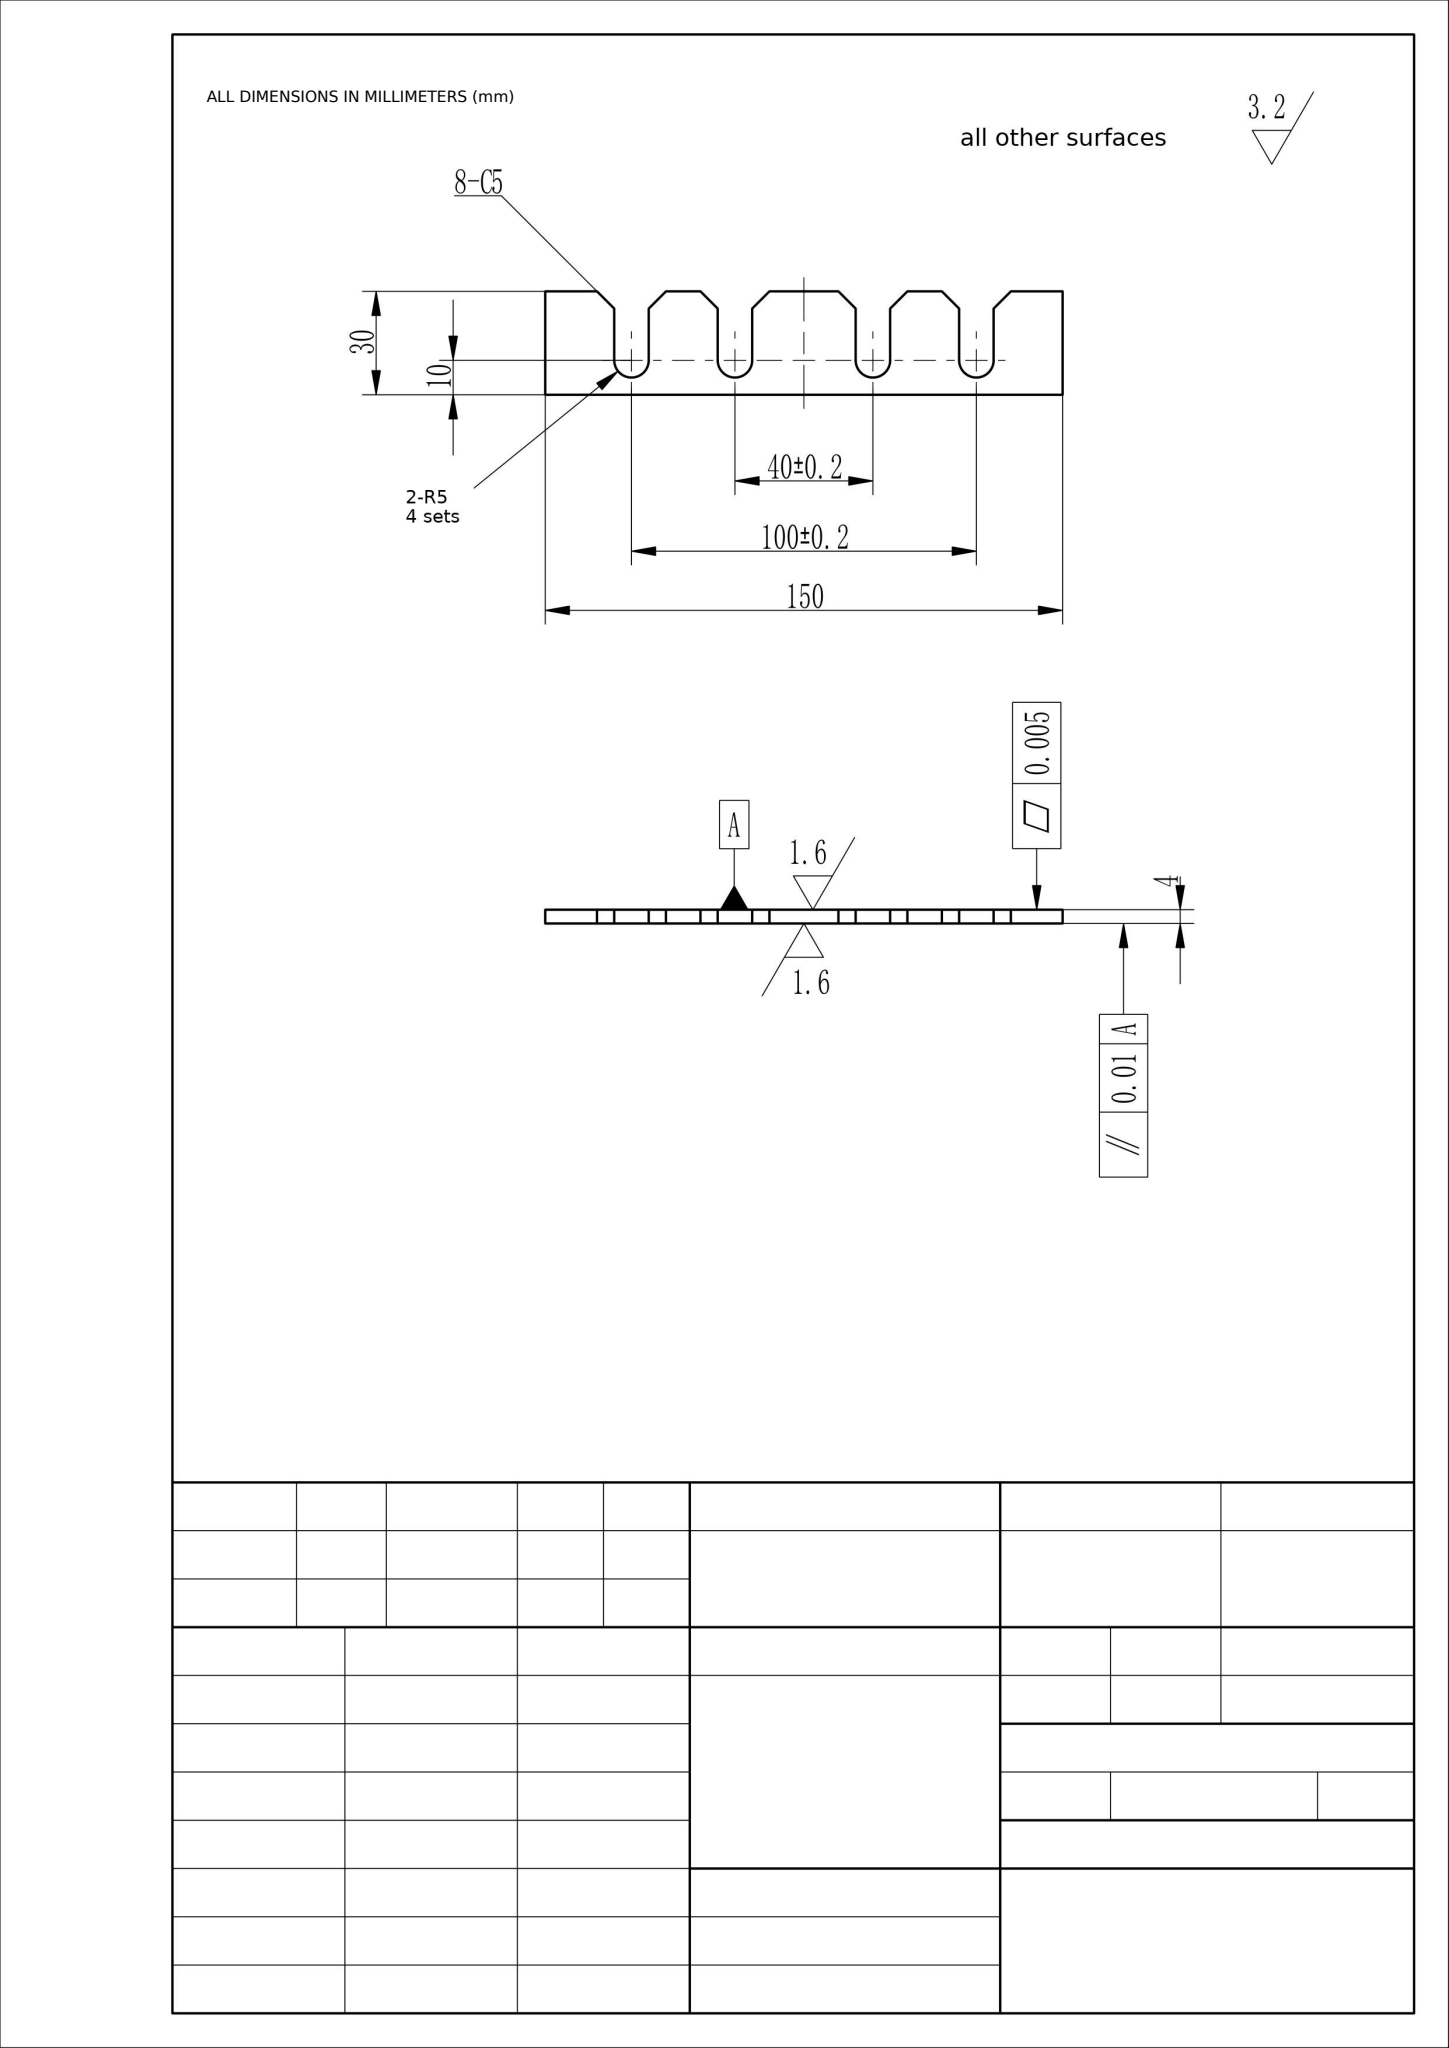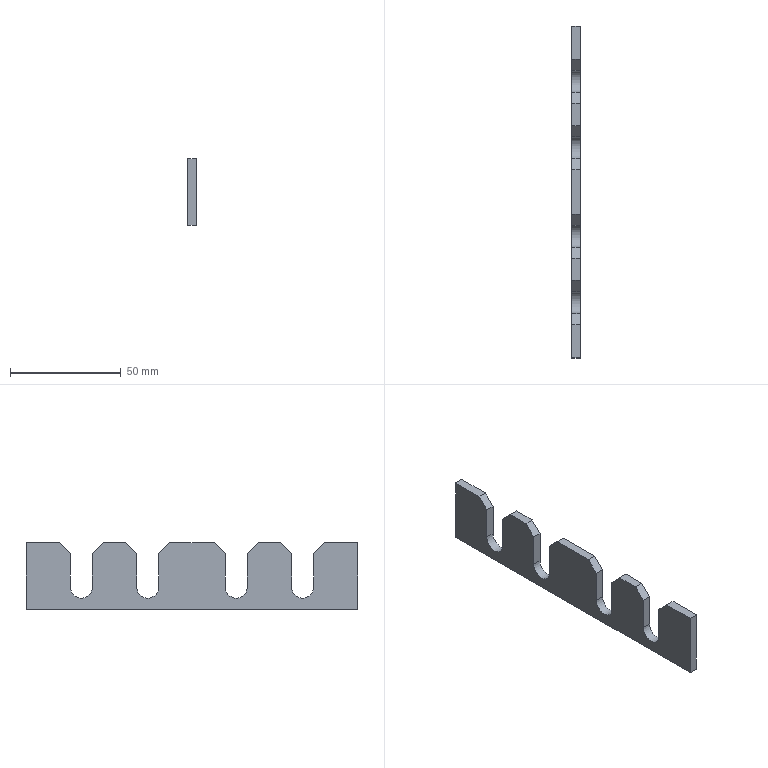Part | NX | mm | 1 solid | 30 faces | box 4 x 150 x 30 mm | volume 13772 mm3 | plane 26 | cylinder 4 | commonest cylinder face diameters 10 x4
STEP:
#1=CARTESIAN_POINT('',(0.,0.,0.));
#2=DIRECTION('',(0.,0.,1.));
#3=DIRECTION('',(1.,0.,0.));
#4=AXIS2_PLACEMENT_3D('',#1,#2,#3);
#5=(LENGTH_UNIT()NAMED_UNIT(*)SI_UNIT(.MILLI.,.METRE.));
#6=UNCERTAINTY_MEASURE_WITH_UNIT(LENGTH_MEASURE(0.00002),#5,'','');
#7=(NAMED_UNIT(*)PLANE_ANGLE_UNIT()SI_UNIT($,.RADIAN.));
#8=PLANE_ANGLE_MEASURE_WITH_UNIT(PLANE_ANGLE_MEASURE(0.01745),#7);
#9=DIMENSIONAL_EXPONENTS(0.,0.,0.,0.,0.,0.,0.);
#10=(CONVERSION_BASED_UNIT('',#8)NAMED_UNIT(#9)PLANE_ANGLE_UNIT());
#11=(NAMED_UNIT(*)SI_UNIT($,.STERADIAN.)SOLID_ANGLE_UNIT());
#12=(GEOMETRIC_REPRESENTATION_CONTEXT(3)GLOBAL_UNCERTAINTY_ASSIGNED_CONTEXT((#6))GLOBAL_UNIT_ASSIGNED_CONTEXT((#5,#10,#11))REPRESENTATION_CONTEXT('',''));
#13=SHAPE_REPRESENTATION('',(#4),#12);
#14=CARTESIAN_POINT('',(4.,-25.,-15.));
#15=VERTEX_POINT('',#14);
#16=CARTESIAN_POINT('',(4.,-25.,0.));
#17=VERTEX_POINT('',#16);
#18=CARTESIAN_POINT('',(4.,-25.,-15.));
#19=DIRECTION('',(0.,-0.,1.));
#20=VECTOR('',#19,1.);
#21=LINE('',#18,#20);
#22=EDGE_CURVE('',#15,#17,#21,.T.);
#23=ORIENTED_EDGE('',*,*,#22,.T.);
#24=CARTESIAN_POINT('',(4.,-30.,5.));
#25=VERTEX_POINT('',#24);
#26=CARTESIAN_POINT('',(4.,-12.5,-12.5));
#27=DIRECTION('',(0.,-0.7071,0.7071));
#28=VECTOR('',#27,1.);
#29=LINE('',#26,#28);
#30=EDGE_CURVE('',#17,#25,#29,.T.);
#31=ORIENTED_EDGE('',*,*,#30,.T.);
#32=CARTESIAN_POINT('',(4.,-40.,5.));
#33=VERTEX_POINT('',#32);
#34=CARTESIAN_POINT('',(4.,75.,5.));
#35=DIRECTION('',(0.,-1.,0.));
#36=VECTOR('',#35,1.);
#37=LINE('',#34,#36);
#38=EDGE_CURVE('',#25,#33,#37,.T.);
#39=ORIENTED_EDGE('',*,*,#38,.T.);
#40=CARTESIAN_POINT('',(4.,-45.,0.));
#41=VERTEX_POINT('',#40);
#42=CARTESIAN_POINT('',(4.,-22.5,22.5));
#43=DIRECTION('',(0.,-0.7071,-0.7071));
#44=VECTOR('',#43,1.);
#45=LINE('',#42,#44);
#46=EDGE_CURVE('',#33,#41,#45,.T.);
#47=ORIENTED_EDGE('',*,*,#46,.T.);
#48=CARTESIAN_POINT('',(4.,-45.,-15.));
#49=VERTEX_POINT('',#48);
#50=CARTESIAN_POINT('',(4.,-45.,35.));
#51=DIRECTION('',(0.,0.,-1.));
#52=VECTOR('',#51,1.);
#53=LINE('',#50,#52);
#54=EDGE_CURVE('',#41,#49,#53,.T.);
#55=ORIENTED_EDGE('',*,*,#54,.T.);
#56=CARTESIAN_POINT('',(4.,-55.,-15.));
#57=VERTEX_POINT('',#56);
#58=CARTESIAN_POINT('',(4.,-50.,-15.));
#59=DIRECTION('',(-1.,0.,0.));
#60=DIRECTION('',(0.,-1.,-0.));
#61=AXIS2_PLACEMENT_3D('',#58,#59,#60);
#62=CIRCLE('',#61,5.);
#63=EDGE_CURVE('',#49,#57,#62,.T.);
#64=ORIENTED_EDGE('',*,*,#63,.T.);
#65=CARTESIAN_POINT('',(4.,-55.,0.));
#66=VERTEX_POINT('',#65);
#67=CARTESIAN_POINT('',(4.,-55.,-15.));
#68=DIRECTION('',(0.,0.,1.));
#69=VECTOR('',#68,1.);
#70=LINE('',#67,#69);
#71=EDGE_CURVE('',#57,#66,#70,.T.);
#72=ORIENTED_EDGE('',*,*,#71,.T.);
#73=CARTESIAN_POINT('',(4.,-60.,5.));
#74=VERTEX_POINT('',#73);
#75=CARTESIAN_POINT('',(4.,-27.5,-27.5));
#76=DIRECTION('',(0.,-0.7071,0.7071));
#77=VECTOR('',#76,1.);
#78=LINE('',#75,#77);
#79=EDGE_CURVE('',#66,#74,#78,.T.);
#80=ORIENTED_EDGE('',*,*,#79,.T.);
#81=CARTESIAN_POINT('',(4.,-75.,5.));
#82=VERTEX_POINT('',#81);
#83=CARTESIAN_POINT('',(4.,75.,5.));
#84=DIRECTION('',(0.,-1.,0.));
#85=VECTOR('',#84,1.);
#86=LINE('',#83,#85);
#87=EDGE_CURVE('',#74,#82,#86,.T.);
#88=ORIENTED_EDGE('',*,*,#87,.T.);
#89=CARTESIAN_POINT('',(4.,-75.,-25.));
#90=VERTEX_POINT('',#89);
#91=CARTESIAN_POINT('',(4.,-75.,25.));
#92=DIRECTION('',(0.,0.,-1.));
#93=VECTOR('',#92,1.);
#94=LINE('',#91,#93);
#95=EDGE_CURVE('',#82,#90,#94,.T.);
#96=ORIENTED_EDGE('',*,*,#95,.T.);
#97=CARTESIAN_POINT('',(4.,75.,-25.));
#98=VERTEX_POINT('',#97);
#99=CARTESIAN_POINT('',(4.,-75.,-25.));
#100=DIRECTION('',(0.,1.,0.));
#101=VECTOR('',#100,1.);
#102=LINE('',#99,#101);
#103=EDGE_CURVE('',#90,#98,#102,.T.);
#104=ORIENTED_EDGE('',*,*,#103,.T.);
#105=CARTESIAN_POINT('',(4.,75.,5.));
#106=VERTEX_POINT('',#105);
#107=CARTESIAN_POINT('',(4.,75.,-25.));
#108=DIRECTION('',(0.,0.,1.));
#109=VECTOR('',#108,1.);
#110=LINE('',#107,#109);
#111=EDGE_CURVE('',#98,#106,#110,.T.);
#112=ORIENTED_EDGE('',*,*,#111,.T.);
#113=CARTESIAN_POINT('',(4.,60.,5.));
#114=VERTEX_POINT('',#113);
#115=CARTESIAN_POINT('',(4.,75.,5.));
#116=DIRECTION('',(0.,-1.,0.));
#117=VECTOR('',#116,1.);
#118=LINE('',#115,#117);
#119=EDGE_CURVE('',#106,#114,#118,.T.);
#120=ORIENTED_EDGE('',*,*,#119,.T.);
#121=CARTESIAN_POINT('',(4.,55.,0.));
#122=VERTEX_POINT('',#121);
#123=CARTESIAN_POINT('',(4.,27.5,-27.5));
#124=DIRECTION('',(0.,-0.7071,-0.7071));
#125=VECTOR('',#124,1.);
#126=LINE('',#123,#125);
#127=EDGE_CURVE('',#114,#122,#126,.T.);
#128=ORIENTED_EDGE('',*,*,#127,.T.);
#129=CARTESIAN_POINT('',(4.,55.,-15.));
#130=VERTEX_POINT('',#129);
#131=CARTESIAN_POINT('',(4.,55.,35.));
#132=DIRECTION('',(0.,0.,-1.));
#133=VECTOR('',#132,1.);
#134=LINE('',#131,#133);
#135=EDGE_CURVE('',#122,#130,#134,.T.);
#136=ORIENTED_EDGE('',*,*,#135,.T.);
#137=CARTESIAN_POINT('',(4.,45.,-15.));
#138=VERTEX_POINT('',#137);
#139=CARTESIAN_POINT('',(4.,50.,-15.));
#140=DIRECTION('',(-1.,0.,0.));
#141=DIRECTION('',(0.,-1.,-0.));
#142=AXIS2_PLACEMENT_3D('',#139,#140,#141);
#143=CIRCLE('',#142,5.);
#144=EDGE_CURVE('',#130,#138,#143,.T.);
#145=ORIENTED_EDGE('',*,*,#144,.T.);
#146=CARTESIAN_POINT('',(4.,45.,0.));
#147=VERTEX_POINT('',#146);
#148=CARTESIAN_POINT('',(4.,45.,-15.));
#149=DIRECTION('',(0.,0.,1.));
#150=VECTOR('',#149,1.);
#151=LINE('',#148,#150);
#152=EDGE_CURVE('',#138,#147,#151,.T.);
#153=ORIENTED_EDGE('',*,*,#152,.T.);
#154=CARTESIAN_POINT('',(4.,40.,5.));
#155=VERTEX_POINT('',#154);
#156=CARTESIAN_POINT('',(4.,22.5,22.5));
#157=DIRECTION('',(0.,-0.7071,0.7071));
#158=VECTOR('',#157,1.);
#159=LINE('',#156,#158);
#160=EDGE_CURVE('',#147,#155,#159,.T.);
#161=ORIENTED_EDGE('',*,*,#160,.T.);
#162=CARTESIAN_POINT('',(4.,30.,5.));
#163=VERTEX_POINT('',#162);
#164=CARTESIAN_POINT('',(4.,75.,5.));
#165=DIRECTION('',(0.,-1.,0.));
#166=VECTOR('',#165,1.);
#167=LINE('',#164,#166);
#168=EDGE_CURVE('',#155,#163,#167,.T.);
#169=ORIENTED_EDGE('',*,*,#168,.T.);
#170=CARTESIAN_POINT('',(4.,25.,0.));
#171=VERTEX_POINT('',#170);
#172=CARTESIAN_POINT('',(4.,12.5,-12.5));
#173=DIRECTION('',(0.,-0.7071,-0.7071));
#174=VECTOR('',#173,1.);
#175=LINE('',#172,#174);
#176=EDGE_CURVE('',#163,#171,#175,.T.);
#177=ORIENTED_EDGE('',*,*,#176,.T.);
#178=CARTESIAN_POINT('',(4.,25.,-15.));
#179=VERTEX_POINT('',#178);
#180=CARTESIAN_POINT('',(4.,25.,35.));
#181=DIRECTION('',(0.,0.,-1.));
#182=VECTOR('',#181,1.);
#183=LINE('',#180,#182);
#184=EDGE_CURVE('',#171,#179,#183,.T.);
#185=ORIENTED_EDGE('',*,*,#184,.T.);
#186=CARTESIAN_POINT('',(4.,15.,-15.));
#187=VERTEX_POINT('',#186);
#188=CARTESIAN_POINT('',(4.,20.,-15.));
#189=DIRECTION('',(-1.,0.,0.));
#190=DIRECTION('',(0.,-1.,-0.));
#191=AXIS2_PLACEMENT_3D('',#188,#189,#190);
#192=CIRCLE('',#191,5.);
#193=EDGE_CURVE('',#179,#187,#192,.T.);
#194=ORIENTED_EDGE('',*,*,#193,.T.);
#195=CARTESIAN_POINT('',(4.,15.,0.));
#196=VERTEX_POINT('',#195);
#197=CARTESIAN_POINT('',(4.,15.,-15.));
#198=DIRECTION('',(0.,-0.,1.));
#199=VECTOR('',#198,1.);
#200=LINE('',#197,#199);
#201=EDGE_CURVE('',#187,#196,#200,.T.);
#202=ORIENTED_EDGE('',*,*,#201,.T.);
#203=CARTESIAN_POINT('',(4.,10.,5.));
#204=VERTEX_POINT('',#203);
#205=CARTESIAN_POINT('',(4.,7.5,7.5));
#206=DIRECTION('',(0.,-0.7071,0.7071));
#207=VECTOR('',#206,1.);
#208=LINE('',#205,#207);
#209=EDGE_CURVE('',#196,#204,#208,.T.);
#210=ORIENTED_EDGE('',*,*,#209,.T.);
#211=CARTESIAN_POINT('',(4.,-10.,5.));
#212=VERTEX_POINT('',#211);
#213=CARTESIAN_POINT('',(4.,75.,5.));
#214=DIRECTION('',(0.,-1.,0.));
#215=VECTOR('',#214,1.);
#216=LINE('',#213,#215);
#217=EDGE_CURVE('',#204,#212,#216,.T.);
#218=ORIENTED_EDGE('',*,*,#217,.T.);
#219=CARTESIAN_POINT('',(4.,-15.,0.));
#220=VERTEX_POINT('',#219);
#221=CARTESIAN_POINT('',(4.,-7.5,7.5));
#222=DIRECTION('',(0.,-0.7071,-0.7071));
#223=VECTOR('',#222,1.);
#224=LINE('',#221,#223);
#225=EDGE_CURVE('',#212,#220,#224,.T.);
#226=ORIENTED_EDGE('',*,*,#225,.T.);
#227=CARTESIAN_POINT('',(4.,-15.,-15.));
#228=VERTEX_POINT('',#227);
#229=CARTESIAN_POINT('',(4.,-15.,35.));
#230=DIRECTION('',(0.,0.,-1.));
#231=VECTOR('',#230,1.);
#232=LINE('',#229,#231);
#233=EDGE_CURVE('',#220,#228,#232,.T.);
#234=ORIENTED_EDGE('',*,*,#233,.T.);
#235=CARTESIAN_POINT('',(4.,-20.,-15.));
#236=DIRECTION('',(-1.,0.,0.));
#237=DIRECTION('',(0.,-1.,-0.));
#238=AXIS2_PLACEMENT_3D('',#235,#236,#237);
#239=CIRCLE('',#238,5.);
#240=EDGE_CURVE('',#228,#15,#239,.T.);
#241=ORIENTED_EDGE('',*,*,#240,.T.);
#242=EDGE_LOOP('',(#23,#31,#39,#47,#55,#64,#72,#80,#88,#96,#104,#112,#120,#128,#136,#145,#153,#161,#169,#177,#185,#194,#202,#210,#218,#226,#234,#241));
#243=FACE_OUTER_BOUND('',#242,.T.);
#244=CARTESIAN_POINT('',(4.,0.,0.));
#245=DIRECTION('',(1.,0.,0.));
#246=DIRECTION('',(0.,0.,-1.));
#247=AXIS2_PLACEMENT_3D('',#244,#245,#246);
#248=PLANE('',#247);
#249=ADVANCED_FACE('',(#243),#248,.T.);
#250=CARTESIAN_POINT('',(0.,-30.,5.));
#251=VERTEX_POINT('',#250);
#252=CARTESIAN_POINT('',(0.,-40.,5.));
#253=VERTEX_POINT('',#252);
#254=CARTESIAN_POINT('',(0.,75.,5.));
#255=DIRECTION('',(0.,-1.,0.));
#256=VECTOR('',#255,1.);
#257=LINE('',#254,#256);
#258=EDGE_CURVE('',#251,#253,#257,.T.);
#259=ORIENTED_EDGE('',*,*,#258,.F.);
#260=CARTESIAN_POINT('',(-0.,-25.,0.));
#261=VERTEX_POINT('',#260);
#262=CARTESIAN_POINT('',(0.,-30.,5.));
#263=DIRECTION('',(0.,0.7071,-0.7071));
#264=VECTOR('',#263,1.);
#265=LINE('',#262,#264);
#266=EDGE_CURVE('',#251,#261,#265,.T.);
#267=ORIENTED_EDGE('',*,*,#266,.T.);
#268=CARTESIAN_POINT('',(-0.,-25.,-15.));
#269=VERTEX_POINT('',#268);
#270=CARTESIAN_POINT('',(-0.,-25.,-15.));
#271=DIRECTION('',(0.,-0.,1.));
#272=VECTOR('',#271,1.);
#273=LINE('',#270,#272);
#274=EDGE_CURVE('',#269,#261,#273,.T.);
#275=ORIENTED_EDGE('',*,*,#274,.F.);
#276=CARTESIAN_POINT('',(-0.,-15.,-15.));
#277=VERTEX_POINT('',#276);
#278=CARTESIAN_POINT('',(-0.,-20.,-15.));
#279=DIRECTION('',(-1.,0.,0.));
#280=DIRECTION('',(0.,-1.,-0.));
#281=AXIS2_PLACEMENT_3D('',#278,#279,#280);
#282=CIRCLE('',#281,5.);
#283=EDGE_CURVE('',#277,#269,#282,.T.);
#284=ORIENTED_EDGE('',*,*,#283,.F.);
#285=CARTESIAN_POINT('',(-0.,-15.,0.));
#286=VERTEX_POINT('',#285);
#287=CARTESIAN_POINT('',(-0.,-15.,35.));
#288=DIRECTION('',(0.,0.,-1.));
#289=VECTOR('',#288,1.);
#290=LINE('',#287,#289);
#291=EDGE_CURVE('',#286,#277,#290,.T.);
#292=ORIENTED_EDGE('',*,*,#291,.F.);
#293=CARTESIAN_POINT('',(0.,-10.,5.));
#294=VERTEX_POINT('',#293);
#295=CARTESIAN_POINT('',(0.,-10.,5.));
#296=DIRECTION('',(0.,0.7071,0.7071));
#297=VECTOR('',#296,1.);
#298=LINE('',#295,#297);
#299=EDGE_CURVE('',#286,#294,#298,.T.);
#300=ORIENTED_EDGE('',*,*,#299,.T.);
#301=CARTESIAN_POINT('',(0.,10.,5.));
#302=VERTEX_POINT('',#301);
#303=CARTESIAN_POINT('',(0.,75.,5.));
#304=DIRECTION('',(0.,-1.,0.));
#305=VECTOR('',#304,1.);
#306=LINE('',#303,#305);
#307=EDGE_CURVE('',#302,#294,#306,.T.);
#308=ORIENTED_EDGE('',*,*,#307,.F.);
#309=CARTESIAN_POINT('',(0.,15.,0.));
#310=VERTEX_POINT('',#309);
#311=CARTESIAN_POINT('',(0.,10.,5.));
#312=DIRECTION('',(0.,0.7071,-0.7071));
#313=VECTOR('',#312,1.);
#314=LINE('',#311,#313);
#315=EDGE_CURVE('',#302,#310,#314,.T.);
#316=ORIENTED_EDGE('',*,*,#315,.T.);
#317=CARTESIAN_POINT('',(0.,15.,-15.));
#318=VERTEX_POINT('',#317);
#319=CARTESIAN_POINT('',(0.,15.,-15.));
#320=DIRECTION('',(0.,-0.,1.));
#321=VECTOR('',#320,1.);
#322=LINE('',#319,#321);
#323=EDGE_CURVE('',#318,#310,#322,.T.);
#324=ORIENTED_EDGE('',*,*,#323,.F.);
#325=CARTESIAN_POINT('',(0.,25.,-15.));
#326=VERTEX_POINT('',#325);
#327=CARTESIAN_POINT('',(0.,20.,-15.));
#328=DIRECTION('',(-1.,0.,0.));
#329=DIRECTION('',(0.,-1.,-0.));
#330=AXIS2_PLACEMENT_3D('',#327,#328,#329);
#331=CIRCLE('',#330,5.);
#332=EDGE_CURVE('',#326,#318,#331,.T.);
#333=ORIENTED_EDGE('',*,*,#332,.F.);
#334=CARTESIAN_POINT('',(0.,25.,0.));
#335=VERTEX_POINT('',#334);
#336=CARTESIAN_POINT('',(0.,25.,35.));
#337=DIRECTION('',(0.,0.,-1.));
#338=VECTOR('',#337,1.);
#339=LINE('',#336,#338);
#340=EDGE_CURVE('',#335,#326,#339,.T.);
#341=ORIENTED_EDGE('',*,*,#340,.F.);
#342=CARTESIAN_POINT('',(0.,30.,5.));
#343=VERTEX_POINT('',#342);
#344=CARTESIAN_POINT('',(0.,30.,5.));
#345=DIRECTION('',(0.,0.7071,0.7071));
#346=VECTOR('',#345,1.);
#347=LINE('',#344,#346);
#348=EDGE_CURVE('',#335,#343,#347,.T.);
#349=ORIENTED_EDGE('',*,*,#348,.T.);
#350=CARTESIAN_POINT('',(0.,40.,5.));
#351=VERTEX_POINT('',#350);
#352=CARTESIAN_POINT('',(0.,75.,5.));
#353=DIRECTION('',(0.,-1.,0.));
#354=VECTOR('',#353,1.);
#355=LINE('',#352,#354);
#356=EDGE_CURVE('',#351,#343,#355,.T.);
#357=ORIENTED_EDGE('',*,*,#356,.F.);
#358=CARTESIAN_POINT('',(0.,45.,0.));
#359=VERTEX_POINT('',#358);
#360=CARTESIAN_POINT('',(0.,40.,5.));
#361=DIRECTION('',(0.,0.7071,-0.7071));
#362=VECTOR('',#361,1.);
#363=LINE('',#360,#362);
#364=EDGE_CURVE('',#351,#359,#363,.T.);
#365=ORIENTED_EDGE('',*,*,#364,.T.);
#366=CARTESIAN_POINT('',(0.,45.,-15.));
#367=VERTEX_POINT('',#366);
#368=CARTESIAN_POINT('',(0.,45.,-15.));
#369=DIRECTION('',(0.,0.,1.));
#370=VECTOR('',#369,1.);
#371=LINE('',#368,#370);
#372=EDGE_CURVE('',#367,#359,#371,.T.);
#373=ORIENTED_EDGE('',*,*,#372,.F.);
#374=CARTESIAN_POINT('',(0.,55.,-15.));
#375=VERTEX_POINT('',#374);
#376=CARTESIAN_POINT('',(0.,50.,-15.));
#377=DIRECTION('',(-1.,0.,0.));
#378=DIRECTION('',(0.,-1.,-0.));
#379=AXIS2_PLACEMENT_3D('',#376,#377,#378);
#380=CIRCLE('',#379,5.);
#381=EDGE_CURVE('',#375,#367,#380,.T.);
#382=ORIENTED_EDGE('',*,*,#381,.F.);
#383=CARTESIAN_POINT('',(0.,55.,0.));
#384=VERTEX_POINT('',#383);
#385=CARTESIAN_POINT('',(0.,55.,35.));
#386=DIRECTION('',(0.,0.,-1.));
#387=VECTOR('',#386,1.);
#388=LINE('',#385,#387);
#389=EDGE_CURVE('',#384,#375,#388,.T.);
#390=ORIENTED_EDGE('',*,*,#389,.F.);
#391=CARTESIAN_POINT('',(0.,60.,5.));
#392=VERTEX_POINT('',#391);
#393=CARTESIAN_POINT('',(0.,60.,5.));
#394=DIRECTION('',(0.,0.7071,0.7071));
#395=VECTOR('',#394,1.);
#396=LINE('',#393,#395);
#397=EDGE_CURVE('',#384,#392,#396,.T.);
#398=ORIENTED_EDGE('',*,*,#397,.T.);
#399=CARTESIAN_POINT('',(0.,75.,5.));
#400=VERTEX_POINT('',#399);
#401=CARTESIAN_POINT('',(0.,75.,5.));
#402=DIRECTION('',(0.,-1.,0.));
#403=VECTOR('',#402,1.);
#404=LINE('',#401,#403);
#405=EDGE_CURVE('',#400,#392,#404,.T.);
#406=ORIENTED_EDGE('',*,*,#405,.F.);
#407=CARTESIAN_POINT('',(0.,75.,-25.));
#408=VERTEX_POINT('',#407);
#409=CARTESIAN_POINT('',(0.,75.,-25.));
#410=DIRECTION('',(0.,0.,1.));
#411=VECTOR('',#410,1.);
#412=LINE('',#409,#411);
#413=EDGE_CURVE('',#408,#400,#412,.T.);
#414=ORIENTED_EDGE('',*,*,#413,.F.);
#415=CARTESIAN_POINT('',(0.,-75.,-25.));
#416=VERTEX_POINT('',#415);
#417=CARTESIAN_POINT('',(0.,-75.,-25.));
#418=DIRECTION('',(0.,1.,0.));
#419=VECTOR('',#418,1.);
#420=LINE('',#417,#419);
#421=EDGE_CURVE('',#416,#408,#420,.T.);
#422=ORIENTED_EDGE('',*,*,#421,.F.);
#423=CARTESIAN_POINT('',(0.,-75.,5.));
#424=VERTEX_POINT('',#423);
#425=CARTESIAN_POINT('',(0.,-75.,25.));
#426=DIRECTION('',(0.,0.,-1.));
#427=VECTOR('',#426,1.);
#428=LINE('',#425,#427);
#429=EDGE_CURVE('',#424,#416,#428,.T.);
#430=ORIENTED_EDGE('',*,*,#429,.F.);
#431=CARTESIAN_POINT('',(0.,-60.,5.));
#432=VERTEX_POINT('',#431);
#433=CARTESIAN_POINT('',(0.,75.,5.));
#434=DIRECTION('',(0.,-1.,0.));
#435=VECTOR('',#434,1.);
#436=LINE('',#433,#435);
#437=EDGE_CURVE('',#432,#424,#436,.T.);
#438=ORIENTED_EDGE('',*,*,#437,.F.);
#439=CARTESIAN_POINT('',(-0.,-55.,0.));
#440=VERTEX_POINT('',#439);
#441=CARTESIAN_POINT('',(0.,-60.,5.));
#442=DIRECTION('',(0.,0.7071,-0.7071));
#443=VECTOR('',#442,1.);
#444=LINE('',#441,#443);
#445=EDGE_CURVE('',#432,#440,#444,.T.);
#446=ORIENTED_EDGE('',*,*,#445,.T.);
#447=CARTESIAN_POINT('',(-0.,-55.,-15.));
#448=VERTEX_POINT('',#447);
#449=CARTESIAN_POINT('',(-0.,-55.,-15.));
#450=DIRECTION('',(0.,0.,1.));
#451=VECTOR('',#450,1.);
#452=LINE('',#449,#451);
#453=EDGE_CURVE('',#448,#440,#452,.T.);
#454=ORIENTED_EDGE('',*,*,#453,.F.);
#455=CARTESIAN_POINT('',(-0.,-45.,-15.));
#456=VERTEX_POINT('',#455);
#457=CARTESIAN_POINT('',(-0.,-50.,-15.));
#458=DIRECTION('',(-1.,0.,0.));
#459=DIRECTION('',(0.,-1.,-0.));
#460=AXIS2_PLACEMENT_3D('',#457,#458,#459);
#461=CIRCLE('',#460,5.);
#462=EDGE_CURVE('',#456,#448,#461,.T.);
#463=ORIENTED_EDGE('',*,*,#462,.F.);
#464=CARTESIAN_POINT('',(-0.,-45.,0.));
#465=VERTEX_POINT('',#464);
#466=CARTESIAN_POINT('',(-0.,-45.,35.));
#467=DIRECTION('',(0.,0.,-1.));
#468=VECTOR('',#467,1.);
#469=LINE('',#466,#468);
#470=EDGE_CURVE('',#465,#456,#469,.T.);
#471=ORIENTED_EDGE('',*,*,#470,.F.);
#472=CARTESIAN_POINT('',(0.,-40.,5.));
#473=DIRECTION('',(0.,0.7071,0.7071));
#474=VECTOR('',#473,1.);
#475=LINE('',#472,#474);
#476=EDGE_CURVE('',#465,#253,#475,.T.);
#477=ORIENTED_EDGE('',*,*,#476,.T.);
#478=EDGE_LOOP('',(#259,#267,#275,#284,#292,#300,#308,#316,#324,#333,#341,#349,#357,#365,#373,#382,#390,#398,#406,#414,#422,#430,#438,#446,#454,#463,#471,#477));
#479=FACE_OUTER_BOUND('',#478,.T.);
#480=CARTESIAN_POINT('',(0.,0.,0.));
#481=DIRECTION('',(1.,0.,0.));
#482=DIRECTION('',(0.,0.,-1.));
#483=AXIS2_PLACEMENT_3D('',#480,#481,#482);
#484=PLANE('',#483);
#485=ADVANCED_FACE('',(#479),#484,.F.);
#486=ORIENTED_EDGE('',*,*,#38,.F.);
#487=CARTESIAN_POINT('',(4.,-30.,5.));
#488=DIRECTION('',(-1.,0.,0.));
#489=VECTOR('',#488,1.);
#490=LINE('',#487,#489);
#491=EDGE_CURVE('',#25,#251,#490,.T.);
#492=ORIENTED_EDGE('',*,*,#491,.T.);
#493=ORIENTED_EDGE('',*,*,#258,.T.);
#494=CARTESIAN_POINT('',(4.,-40.,5.));
#495=DIRECTION('',(1.,0.,0.));
#496=VECTOR('',#495,1.);
#497=LINE('',#494,#496);
#498=EDGE_CURVE('',#253,#33,#497,.T.);
#499=ORIENTED_EDGE('',*,*,#498,.T.);
#500=EDGE_LOOP('',(#486,#492,#493,#499));
#501=FACE_OUTER_BOUND('',#500,.T.);
#502=CARTESIAN_POINT('',(4.,75.,5.));
#503=DIRECTION('',(0.,0.,-1.));
#504=DIRECTION('',(-1.,0.,0.));
#505=AXIS2_PLACEMENT_3D('',#502,#503,#504);
#506=PLANE('',#505);
#507=ADVANCED_FACE('',(#501),#506,.F.);
#508=ORIENTED_EDGE('',*,*,#307,.T.);
#509=CARTESIAN_POINT('',(4.,-10.,5.));
#510=DIRECTION('',(1.,0.,0.));
#511=VECTOR('',#510,1.);
#512=LINE('',#509,#511);
#513=EDGE_CURVE('',#294,#212,#512,.T.);
#514=ORIENTED_EDGE('',*,*,#513,.T.);
#515=ORIENTED_EDGE('',*,*,#217,.F.);
#516=CARTESIAN_POINT('',(4.,10.,5.));
#517=DIRECTION('',(-1.,0.,0.));
#518=VECTOR('',#517,1.);
#519=LINE('',#516,#518);
#520=EDGE_CURVE('',#204,#302,#519,.T.);
#521=ORIENTED_EDGE('',*,*,#520,.T.);
#522=EDGE_LOOP('',(#508,#514,#515,#521));
#523=FACE_OUTER_BOUND('',#522,.T.);
#524=CARTESIAN_POINT('',(4.,75.,5.));
#525=DIRECTION('',(0.,0.,-1.));
#526=DIRECTION('',(-1.,0.,0.));
#527=AXIS2_PLACEMENT_3D('',#524,#525,#526);
#528=PLANE('',#527);
#529=ADVANCED_FACE('',(#523),#528,.F.);
#530=ORIENTED_EDGE('',*,*,#87,.F.);
#531=CARTESIAN_POINT('',(4.,-60.,5.));
#532=DIRECTION('',(-1.,0.,0.));
#533=VECTOR('',#532,1.);
#534=LINE('',#531,#533);
#535=EDGE_CURVE('',#74,#432,#534,.T.);
#536=ORIENTED_EDGE('',*,*,#535,.T.);
#537=ORIENTED_EDGE('',*,*,#437,.T.);
#538=CARTESIAN_POINT('',(4.,-75.,5.));
#539=DIRECTION('',(-1.,0.,0.));
#540=VECTOR('',#539,1.);
#541=LINE('',#538,#540);
#542=EDGE_CURVE('',#82,#424,#541,.T.);
#543=ORIENTED_EDGE('',*,*,#542,.F.);
#544=EDGE_LOOP('',(#530,#536,#537,#543));
#545=FACE_OUTER_BOUND('',#544,.T.);
#546=CARTESIAN_POINT('',(4.,75.,5.));
#547=DIRECTION('',(0.,0.,-1.));
#548=DIRECTION('',(-1.,0.,0.));
#549=AXIS2_PLACEMENT_3D('',#546,#547,#548);
#550=PLANE('',#549);
#551=ADVANCED_FACE('',(#545),#550,.F.);
#552=ORIENTED_EDGE('',*,*,#356,.T.);
#553=CARTESIAN_POINT('',(4.,30.,5.));
#554=DIRECTION('',(1.,0.,0.));
#555=VECTOR('',#554,1.);
#556=LINE('',#553,#555);
#557=EDGE_CURVE('',#343,#163,#556,.T.);
#558=ORIENTED_EDGE('',*,*,#557,.T.);
#559=ORIENTED_EDGE('',*,*,#168,.F.);
#560=CARTESIAN_POINT('',(4.,40.,5.));
#561=DIRECTION('',(-1.,0.,0.));
#562=VECTOR('',#561,1.);
#563=LINE('',#560,#562);
#564=EDGE_CURVE('',#155,#351,#563,.T.);
#565=ORIENTED_EDGE('',*,*,#564,.T.);
#566=EDGE_LOOP('',(#552,#558,#559,#565));
#567=FACE_OUTER_BOUND('',#566,.T.);
#568=CARTESIAN_POINT('',(4.,75.,5.));
#569=DIRECTION('',(0.,0.,-1.));
#570=DIRECTION('',(-1.,0.,0.));
#571=AXIS2_PLACEMENT_3D('',#568,#569,#570);
#572=PLANE('',#571);
#573=ADVANCED_FACE('',(#567),#572,.F.);
#574=ORIENTED_EDGE('',*,*,#429,.T.);
#575=CARTESIAN_POINT('',(4.,-75.,-25.));
#576=DIRECTION('',(-1.,0.,0.));
#577=VECTOR('',#576,1.);
#578=LINE('',#575,#577);
#579=EDGE_CURVE('',#90,#416,#578,.T.);
#580=ORIENTED_EDGE('',*,*,#579,.F.);
#581=ORIENTED_EDGE('',*,*,#95,.F.);
#582=ORIENTED_EDGE('',*,*,#542,.T.);
#583=EDGE_LOOP('',(#574,#580,#581,#582));
#584=FACE_OUTER_BOUND('',#583,.T.);
#585=CARTESIAN_POINT('',(4.,-75.,25.));
#586=DIRECTION('',(0.,1.,0.));
#587=DIRECTION('',(0.,0.,1.));
#588=AXIS2_PLACEMENT_3D('',#585,#586,#587);
#589=PLANE('',#588);
#590=ADVANCED_FACE('',(#584),#589,.F.);
#591=ORIENTED_EDGE('',*,*,#421,.T.);
#592=CARTESIAN_POINT('',(4.,75.,-25.));
#593=DIRECTION('',(-1.,0.,0.));
#594=VECTOR('',#593,1.);
#595=LINE('',#592,#594);
#596=EDGE_CURVE('',#98,#408,#595,.T.);
#597=ORIENTED_EDGE('',*,*,#596,.F.);
#598=ORIENTED_EDGE('',*,*,#103,.F.);
#599=ORIENTED_EDGE('',*,*,#579,.T.);
#600=EDGE_LOOP('',(#591,#597,#598,#599));
#601=FACE_OUTER_BOUND('',#600,.T.);
#602=CARTESIAN_POINT('',(4.,-75.,-25.));
#603=DIRECTION('',(0.,0.,1.));
#604=DIRECTION('',(1.,0.,0.));
#605=AXIS2_PLACEMENT_3D('',#602,#603,#604);
#606=PLANE('',#605);
#607=ADVANCED_FACE('',(#601),#606,.F.);
#608=ORIENTED_EDGE('',*,*,#413,.T.);
#609=CARTESIAN_POINT('',(4.,75.,5.));
#610=DIRECTION('',(-1.,0.,0.));
#611=VECTOR('',#610,1.);
#612=LINE('',#609,#611);
#613=EDGE_CURVE('',#106,#400,#612,.T.);
#614=ORIENTED_EDGE('',*,*,#613,.F.);
#615=ORIENTED_EDGE('',*,*,#111,.F.);
#616=ORIENTED_EDGE('',*,*,#596,.T.);
#617=EDGE_LOOP('',(#608,#614,#615,#616));
#618=FACE_OUTER_BOUND('',#617,.T.);
#619=CARTESIAN_POINT('',(4.,75.,-25.));
#620=DIRECTION('',(0.,-1.,0.));
#621=DIRECTION('',(0.,0.,-1.));
#622=AXIS2_PLACEMENT_3D('',#619,#620,#621);
#623=PLANE('',#622);
#624=ADVANCED_FACE('',(#618),#623,.F.);
#625=ORIENTED_EDGE('',*,*,#405,.T.);
#626=CARTESIAN_POINT('',(4.,60.,5.));
#627=DIRECTION('',(1.,0.,0.));
#628=VECTOR('',#627,1.);
#629=LINE('',#626,#628);
#630=EDGE_CURVE('',#392,#114,#629,.T.);
#631=ORIENTED_EDGE('',*,*,#630,.T.);
#632=ORIENTED_EDGE('',*,*,#119,.F.);
#633=ORIENTED_EDGE('',*,*,#613,.T.);
#634=EDGE_LOOP('',(#625,#631,#632,#633));
#635=FACE_OUTER_BOUND('',#634,.T.);
#636=CARTESIAN_POINT('',(4.,75.,5.));
#637=DIRECTION('',(0.,0.,-1.));
#638=DIRECTION('',(-1.,0.,0.));
#639=AXIS2_PLACEMENT_3D('',#636,#637,#638);
#640=PLANE('',#639);
#641=ADVANCED_FACE('',(#635),#640,.F.);
#642=ORIENTED_EDGE('',*,*,#372,.T.);
#643=CARTESIAN_POINT('',(4.,45.,0.));
#644=DIRECTION('',(1.,0.,0.));
#645=VECTOR('',#644,1.);
#646=LINE('',#643,#645);
#647=EDGE_CURVE('',#359,#147,#646,.T.);
#648=ORIENTED_EDGE('',*,*,#647,.T.);
#649=ORIENTED_EDGE('',*,*,#152,.F.);
#650=CARTESIAN_POINT('',(4.,45.,-15.));
#651=DIRECTION('',(1.,0.,0.));
#652=VECTOR('',#651,1.);
#653=LINE('',#650,#652);
#654=EDGE_CURVE('',#367,#138,#653,.T.);
#655=ORIENTED_EDGE('',*,*,#654,.F.);
#656=EDGE_LOOP('',(#642,#648,#649,#655));
#657=FACE_OUTER_BOUND('',#656,.T.);
#658=CARTESIAN_POINT('',(4.,45.,-15.));
#659=DIRECTION('',(0.,-1.,0.));
#660=DIRECTION('',(0.,0.,-1.));
#661=AXIS2_PLACEMENT_3D('',#658,#659,#660);
#662=PLANE('',#661);
#663=ADVANCED_FACE('',(#657),#662,.F.);
#664=ORIENTED_EDGE('',*,*,#135,.F.);
#665=CARTESIAN_POINT('',(4.,55.,0.));
#666=DIRECTION('',(-1.,0.,0.));
#667=VECTOR('',#666,1.);
#668=LINE('',#665,#667);
#669=EDGE_CURVE('',#122,#384,#668,.T.);
#670=ORIENTED_EDGE('',*,*,#669,.T.);
#671=ORIENTED_EDGE('',*,*,#389,.T.);
#672=CARTESIAN_POINT('',(4.,55.,-15.));
#673=DIRECTION('',(1.,0.,0.));
#674=VECTOR('',#673,1.);
#675=LINE('',#672,#674);
#676=EDGE_CURVE('',#375,#130,#675,.T.);
#677=ORIENTED_EDGE('',*,*,#676,.T.);
#678=EDGE_LOOP('',(#664,#670,#671,#677));
#679=FACE_OUTER_BOUND('',#678,.T.);
#680=CARTESIAN_POINT('',(4.,55.,35.));
#681=DIRECTION('',(0.,1.,0.));
#682=DIRECTION('',(0.,0.,1.));
#683=AXIS2_PLACEMENT_3D('',#680,#681,#682);
#684=PLANE('',#683);
#685=ADVANCED_FACE('',(#679),#684,.F.);
#686=ORIENTED_EDGE('',*,*,#381,.T.);
#687=ORIENTED_EDGE('',*,*,#654,.T.);
#688=ORIENTED_EDGE('',*,*,#144,.F.);
#689=ORIENTED_EDGE('',*,*,#676,.F.);
#690=EDGE_LOOP('',(#686,#687,#688,#689));
#691=FACE_OUTER_BOUND('',#690,.T.);
#692=CARTESIAN_POINT('',(4.,50.,-15.));
#693=DIRECTION('',(-1.,0.,0.));
#694=DIRECTION('',(0.,0.,1.));
#695=AXIS2_PLACEMENT_3D('',#692,#693,#694);
#696=CYLINDRICAL_SURFACE('',#695,5.);
#697=ADVANCED_FACE('',(#691),#696,.F.);
#698=ORIENTED_EDGE('',*,*,#453,.T.);
#699=CARTESIAN_POINT('',(4.,-55.,0.));
#700=DIRECTION('',(1.,0.,0.));
#701=VECTOR('',#700,1.);
#702=LINE('',#699,#701);
#703=EDGE_CURVE('',#440,#66,#702,.T.);
#704=ORIENTED_EDGE('',*,*,#703,.T.);
#705=ORIENTED_EDGE('',*,*,#71,.F.);
#706=CARTESIAN_POINT('',(4.,-55.,-15.));
#707=DIRECTION('',(1.,0.,0.));
#708=VECTOR('',#707,1.);
#709=LINE('',#706,#708);
#710=EDGE_CURVE('',#448,#57,#709,.T.);
#711=ORIENTED_EDGE('',*,*,#710,.F.);
#712=EDGE_LOOP('',(#698,#704,#705,#711));
#713=FACE_OUTER_BOUND('',#712,.T.);
#714=CARTESIAN_POINT('',(4.,-55.,-15.));
#715=DIRECTION('',(0.,-1.,0.));
#716=DIRECTION('',(0.,0.,-1.));
#717=AXIS2_PLACEMENT_3D('',#714,#715,#716);
#718=PLANE('',#717);
#719=ADVANCED_FACE('',(#713),#718,.F.);
#720=ORIENTED_EDGE('',*,*,#54,.F.);
#721=CARTESIAN_POINT('',(4.,-45.,0.));
#722=DIRECTION('',(-1.,0.,0.));
#723=VECTOR('',#722,1.);
#724=LINE('',#721,#723);
#725=EDGE_CURVE('',#41,#465,#724,.T.);
#726=ORIENTED_EDGE('',*,*,#725,.T.);
#727=ORIENTED_EDGE('',*,*,#470,.T.);
#728=CARTESIAN_POINT('',(4.,-45.,-15.));
#729=DIRECTION('',(1.,0.,0.));
#730=VECTOR('',#729,1.);
#731=LINE('',#728,#730);
#732=EDGE_CURVE('',#456,#49,#731,.T.);
#733=ORIENTED_EDGE('',*,*,#732,.T.);
#734=EDGE_LOOP('',(#720,#726,#727,#733));
#735=FACE_OUTER_BOUND('',#734,.T.);
#736=CARTESIAN_POINT('',(4.,-45.,35.));
#737=DIRECTION('',(0.,1.,0.));
#738=DIRECTION('',(0.,0.,1.));
#739=AXIS2_PLACEMENT_3D('',#736,#737,#738);
#740=PLANE('',#739);
#741=ADVANCED_FACE('',(#735),#740,.F.);
#742=ORIENTED_EDGE('',*,*,#462,.T.);
#743=ORIENTED_EDGE('',*,*,#710,.T.);
#744=ORIENTED_EDGE('',*,*,#63,.F.);
#745=ORIENTED_EDGE('',*,*,#732,.F.);
#746=EDGE_LOOP('',(#742,#743,#744,#745));
#747=FACE_OUTER_BOUND('',#746,.T.);
#748=CARTESIAN_POINT('',(4.,-50.,-15.));
#749=DIRECTION('',(-1.,0.,0.));
#750=DIRECTION('',(0.,0.,1.));
#751=AXIS2_PLACEMENT_3D('',#748,#749,#750);
#752=CYLINDRICAL_SURFACE('',#751,5.);
#753=ADVANCED_FACE('',(#747),#752,.F.);
#754=ORIENTED_EDGE('',*,*,#79,.F.);
#755=ORIENTED_EDGE('',*,*,#703,.F.);
#756=ORIENTED_EDGE('',*,*,#445,.F.);
#757=ORIENTED_EDGE('',*,*,#535,.F.);
#758=EDGE_LOOP('',(#754,#755,#756,#757));
#759=FACE_OUTER_BOUND('',#758,.T.);
#760=CARTESIAN_POINT('',(4.,-60.,5.));
#761=DIRECTION('',(0.,-0.7071,-0.7071));
#762=DIRECTION('',(0.,0.7071,-0.7071));
#763=AXIS2_PLACEMENT_3D('',#760,#761,#762);
#764=PLANE('',#763);
#765=ADVANCED_FACE('',(#759),#764,.F.);
#766=ORIENTED_EDGE('',*,*,#476,.F.);
#767=ORIENTED_EDGE('',*,*,#725,.F.);
#768=ORIENTED_EDGE('',*,*,#46,.F.);
#769=ORIENTED_EDGE('',*,*,#498,.F.);
#770=EDGE_LOOP('',(#766,#767,#768,#769));
#771=FACE_OUTER_BOUND('',#770,.T.);
#772=CARTESIAN_POINT('',(4.,-40.,5.));
#773=DIRECTION('',(0.,0.7071,-0.7071));
#774=DIRECTION('',(0.,0.7071,0.7071));
#775=AXIS2_PLACEMENT_3D('',#772,#773,#774);
#776=PLANE('',#775);
#777=ADVANCED_FACE('',(#771),#776,.F.);
#778=ORIENTED_EDGE('',*,*,#160,.F.);
#779=ORIENTED_EDGE('',*,*,#647,.F.);
#780=ORIENTED_EDGE('',*,*,#364,.F.);
#781=ORIENTED_EDGE('',*,*,#564,.F.);
#782=EDGE_LOOP('',(#778,#779,#780,#781));
#783=FACE_OUTER_BOUND('',#782,.T.);
#784=CARTESIAN_POINT('',(4.,40.,5.));
#785=DIRECTION('',(0.,-0.7071,-0.7071));
#786=DIRECTION('',(0.,0.7071,-0.7071));
#787=AXIS2_PLACEMENT_3D('',#784,#785,#786);
#788=PLANE('',#787);
#789=ADVANCED_FACE('',(#783),#788,.F.);
#790=ORIENTED_EDGE('',*,*,#397,.F.);
#791=ORIENTED_EDGE('',*,*,#669,.F.);
#792=ORIENTED_EDGE('',*,*,#127,.F.);
#793=ORIENTED_EDGE('',*,*,#630,.F.);
#794=EDGE_LOOP('',(#790,#791,#792,#793));
#795=FACE_OUTER_BOUND('',#794,.T.);
#796=CARTESIAN_POINT('',(4.,60.,5.));
#797=DIRECTION('',(0.,0.7071,-0.7071));
#798=DIRECTION('',(0.,0.7071,0.7071));
#799=AXIS2_PLACEMENT_3D('',#796,#797,#798);
#800=PLANE('',#799);
#801=ADVANCED_FACE('',(#795),#800,.F.);
#802=ORIENTED_EDGE('',*,*,#323,.T.);
#803=CARTESIAN_POINT('',(4.,15.,0.));
#804=DIRECTION('',(1.,0.,0.));
#805=VECTOR('',#804,1.);
#806=LINE('',#803,#805);
#807=EDGE_CURVE('',#310,#196,#806,.T.);
#808=ORIENTED_EDGE('',*,*,#807,.T.);
#809=ORIENTED_EDGE('',*,*,#201,.F.);
#810=CARTESIAN_POINT('',(4.,15.,-15.));
#811=DIRECTION('',(1.,0.,0.));
#812=VECTOR('',#811,1.);
#813=LINE('',#810,#812);
#814=EDGE_CURVE('',#318,#187,#813,.T.);
#815=ORIENTED_EDGE('',*,*,#814,.F.);
#816=EDGE_LOOP('',(#802,#808,#809,#815));
#817=FACE_OUTER_BOUND('',#816,.T.);
#818=CARTESIAN_POINT('',(4.,15.,-15.));
#819=DIRECTION('',(0.,-1.,-0.));
#820=DIRECTION('',(0.,0.,-1.));
#821=AXIS2_PLACEMENT_3D('',#818,#819,#820);
#822=PLANE('',#821);
#823=ADVANCED_FACE('',(#817),#822,.F.);
#824=ORIENTED_EDGE('',*,*,#184,.F.);
#825=CARTESIAN_POINT('',(4.,25.,0.));
#826=DIRECTION('',(-1.,0.,0.));
#827=VECTOR('',#826,1.);
#828=LINE('',#825,#827);
#829=EDGE_CURVE('',#171,#335,#828,.T.);
#830=ORIENTED_EDGE('',*,*,#829,.T.);
#831=ORIENTED_EDGE('',*,*,#340,.T.);
#832=CARTESIAN_POINT('',(4.,25.,-15.));
#833=DIRECTION('',(1.,0.,0.));
#834=VECTOR('',#833,1.);
#835=LINE('',#832,#834);
#836=EDGE_CURVE('',#326,#179,#835,.T.);
#837=ORIENTED_EDGE('',*,*,#836,.T.);
#838=EDGE_LOOP('',(#824,#830,#831,#837));
#839=FACE_OUTER_BOUND('',#838,.T.);
#840=CARTESIAN_POINT('',(4.,25.,35.));
#841=DIRECTION('',(0.,1.,0.));
#842=DIRECTION('',(0.,-0.,1.));
#843=AXIS2_PLACEMENT_3D('',#840,#841,#842);
#844=PLANE('',#843);
#845=ADVANCED_FACE('',(#839),#844,.F.);
#846=ORIENTED_EDGE('',*,*,#332,.T.);
#847=ORIENTED_EDGE('',*,*,#814,.T.);
#848=ORIENTED_EDGE('',*,*,#193,.F.);
#849=ORIENTED_EDGE('',*,*,#836,.F.);
#850=EDGE_LOOP('',(#846,#847,#848,#849));
#851=FACE_OUTER_BOUND('',#850,.T.);
#852=CARTESIAN_POINT('',(4.,20.,-15.));
#853=DIRECTION('',(-1.,0.,0.));
#854=DIRECTION('',(0.,0.,1.));
#855=AXIS2_PLACEMENT_3D('',#852,#853,#854);
#856=CYLINDRICAL_SURFACE('',#855,5.);
#857=ADVANCED_FACE('',(#851),#856,.F.);
#858=ORIENTED_EDGE('',*,*,#274,.T.);
#859=CARTESIAN_POINT('',(4.,-25.,0.));
#860=DIRECTION('',(1.,0.,0.));
#861=VECTOR('',#860,1.);
#862=LINE('',#859,#861);
#863=EDGE_CURVE('',#261,#17,#862,.T.);
#864=ORIENTED_EDGE('',*,*,#863,.T.);
#865=ORIENTED_EDGE('',*,*,#22,.F.);
#866=CARTESIAN_POINT('',(4.,-25.,-15.));
#867=DIRECTION('',(1.,0.,0.));
#868=VECTOR('',#867,1.);
#869=LINE('',#866,#868);
#870=EDGE_CURVE('',#269,#15,#869,.T.);
#871=ORIENTED_EDGE('',*,*,#870,.F.);
#872=EDGE_LOOP('',(#858,#864,#865,#871));
#873=FACE_OUTER_BOUND('',#872,.T.);
#874=CARTESIAN_POINT('',(4.,-25.,-15.));
#875=DIRECTION('',(0.,-1.,-0.));
#876=DIRECTION('',(0.,0.,-1.));
#877=AXIS2_PLACEMENT_3D('',#874,#875,#876);
#878=PLANE('',#877);
#879=ADVANCED_FACE('',(#873),#878,.F.);
#880=ORIENTED_EDGE('',*,*,#233,.F.);
#881=CARTESIAN_POINT('',(4.,-15.,0.));
#882=DIRECTION('',(-1.,0.,0.));
#883=VECTOR('',#882,1.);
#884=LINE('',#881,#883);
#885=EDGE_CURVE('',#220,#286,#884,.T.);
#886=ORIENTED_EDGE('',*,*,#885,.T.);
#887=ORIENTED_EDGE('',*,*,#291,.T.);
#888=CARTESIAN_POINT('',(4.,-15.,-15.));
#889=DIRECTION('',(1.,0.,0.));
#890=VECTOR('',#889,1.);
#891=LINE('',#888,#890);
#892=EDGE_CURVE('',#277,#228,#891,.T.);
#893=ORIENTED_EDGE('',*,*,#892,.T.);
#894=EDGE_LOOP('',(#880,#886,#887,#893));
#895=FACE_OUTER_BOUND('',#894,.T.);
#896=CARTESIAN_POINT('',(4.,-15.,35.));
#897=DIRECTION('',(0.,1.,0.));
#898=DIRECTION('',(0.,-0.,1.));
#899=AXIS2_PLACEMENT_3D('',#896,#897,#898);
#900=PLANE('',#899);
#901=ADVANCED_FACE('',(#895),#900,.F.);
#902=ORIENTED_EDGE('',*,*,#283,.T.);
#903=ORIENTED_EDGE('',*,*,#870,.T.);
#904=ORIENTED_EDGE('',*,*,#240,.F.);
#905=ORIENTED_EDGE('',*,*,#892,.F.);
#906=EDGE_LOOP('',(#902,#903,#904,#905));
#907=FACE_OUTER_BOUND('',#906,.T.);
#908=CARTESIAN_POINT('',(4.,-20.,-15.));
#909=DIRECTION('',(-1.,0.,0.));
#910=DIRECTION('',(0.,0.,1.));
#911=AXIS2_PLACEMENT_3D('',#908,#909,#910);
#912=CYLINDRICAL_SURFACE('',#911,5.);
#913=ADVANCED_FACE('',(#907),#912,.F.);
#914=ORIENTED_EDGE('',*,*,#30,.F.);
#915=ORIENTED_EDGE('',*,*,#863,.F.);
#916=ORIENTED_EDGE('',*,*,#266,.F.);
#917=ORIENTED_EDGE('',*,*,#491,.F.);
#918=EDGE_LOOP('',(#914,#915,#916,#917));
#919=FACE_OUTER_BOUND('',#918,.T.);
#920=CARTESIAN_POINT('',(4.,-30.,5.));
#921=DIRECTION('',(0.,-0.7071,-0.7071));
#922=DIRECTION('',(0.,0.7071,-0.7071));
#923=AXIS2_PLACEMENT_3D('',#920,#921,#922);
#924=PLANE('',#923);
#925=ADVANCED_FACE('',(#919),#924,.F.);
#926=ORIENTED_EDGE('',*,*,#299,.F.);
#927=ORIENTED_EDGE('',*,*,#885,.F.);
#928=ORIENTED_EDGE('',*,*,#225,.F.);
#929=ORIENTED_EDGE('',*,*,#513,.F.);
#930=EDGE_LOOP('',(#926,#927,#928,#929));
#931=FACE_OUTER_BOUND('',#930,.T.);
#932=CARTESIAN_POINT('',(4.,-10.,5.));
#933=DIRECTION('',(0.,0.7071,-0.7071));
#934=DIRECTION('',(0.,0.7071,0.7071));
#935=AXIS2_PLACEMENT_3D('',#932,#933,#934);
#936=PLANE('',#935);
#937=ADVANCED_FACE('',(#931),#936,.F.);
#938=ORIENTED_EDGE('',*,*,#209,.F.);
#939=ORIENTED_EDGE('',*,*,#807,.F.);
#940=ORIENTED_EDGE('',*,*,#315,.F.);
#941=ORIENTED_EDGE('',*,*,#520,.F.);
#942=EDGE_LOOP('',(#938,#939,#940,#941));
#943=FACE_OUTER_BOUND('',#942,.T.);
#944=CARTESIAN_POINT('',(4.,10.,5.));
#945=DIRECTION('',(0.,-0.7071,-0.7071));
#946=DIRECTION('',(0.,0.7071,-0.7071));
#947=AXIS2_PLACEMENT_3D('',#944,#945,#946);
#948=PLANE('',#947);
#949=ADVANCED_FACE('',(#943),#948,.F.);
#950=ORIENTED_EDGE('',*,*,#348,.F.);
#951=ORIENTED_EDGE('',*,*,#829,.F.);
#952=ORIENTED_EDGE('',*,*,#176,.F.);
#953=ORIENTED_EDGE('',*,*,#557,.F.);
#954=EDGE_LOOP('',(#950,#951,#952,#953));
#955=FACE_OUTER_BOUND('',#954,.T.);
#956=CARTESIAN_POINT('',(4.,30.,5.));
#957=DIRECTION('',(0.,0.7071,-0.7071));
#958=DIRECTION('',(0.,0.7071,0.7071));
#959=AXIS2_PLACEMENT_3D('',#956,#957,#958);
#960=PLANE('',#959);
#961=ADVANCED_FACE('',(#955),#960,.F.);
#962=CLOSED_SHELL('',(#249,#485,#507,#529,#551,#573,#590,#607,#624,#641,#663,#685,#697,#719,#741,#753,#765,#777,#789,#801,#823,#845,#857,#879,#901,#913,#925,#937,#949,#961));
#963=MANIFOLD_SOLID_BREP('',#962);
#964=ADVANCED_BREP_SHAPE_REPRESENTATION('',(#963),#12);
#965=SHAPE_REPRESENTATION_RELATIONSHIP('','',#13,#964);
#966=PRESENTATION_LAYER_ASSIGNMENT('','',(#963));
#967=COLOUR_RGB('',1.,0.6,0.);
#968=FILL_AREA_STYLE_COLOUR('',#967);
#969=FILL_AREA_STYLE('',(#968));
#970=SURFACE_STYLE_FILL_AREA(#969);
#971=SURFACE_SIDE_STYLE('',(#970));
#972=SURFACE_STYLE_USAGE(.BOTH.,#971);
#973=PRESENTATION_STYLE_ASSIGNMENT((#972));
#974=STYLED_ITEM('',(#973),#963);
#975=MECHANICAL_DESIGN_GEOMETRIC_PRESENTATION_REPRESENTATION('',(#974),#12);